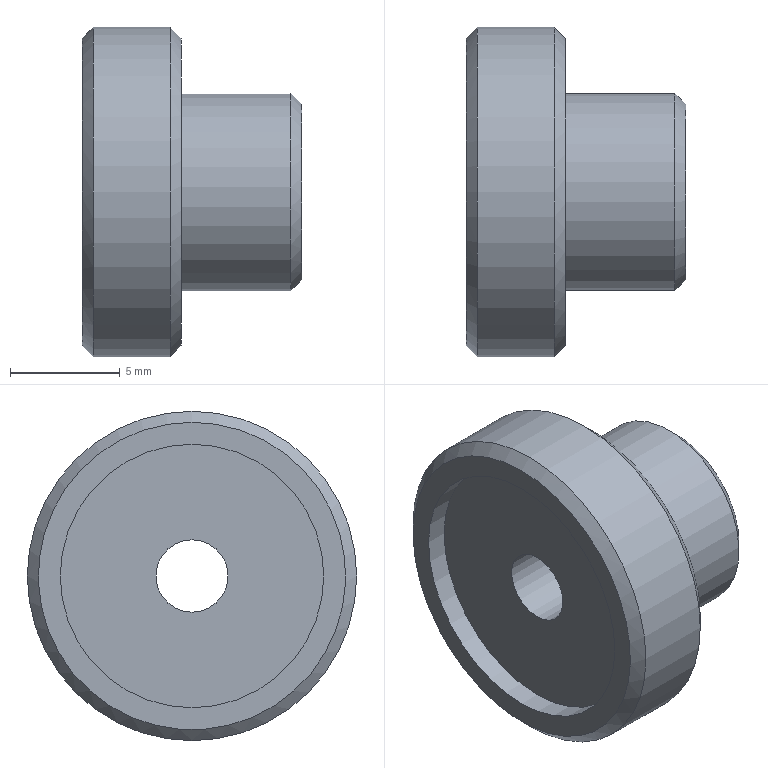Component | NX | 2_KNURLED_NUT | 1 solid | 11 faces | box 10 x 15 x 15 mm | volume 940 mm3 | plane 4 | cylinder 4 | cone 3 | commonest cylinder face diameters 15 x1 9 x1 3.3 x1 12 x1
STEP:
#1=CARTESIAN_POINT('',(0.,0.,0.));
#2=DIRECTION('',(0.,0.,1.));
#3=DIRECTION('',(1.,0.,0.));
#4=AXIS2_PLACEMENT_3D('',#1,#2,#3);
#5=CARTESIAN_POINT('',(-76.584,-174.206,-245.219));
#6=VERTEX_POINT('',#5);
#7=CARTESIAN_POINT('',(-76.584,-174.206,-238.219));
#8=DIRECTION('',(1.,0.,0.));
#9=DIRECTION('',(0.,0.,-1.));
#10=AXIS2_PLACEMENT_3D('',#7,#8,#9);
#11=CIRCLE('',#10,7.);
#12=CARTESIAN_POINT('',(-76.584,-174.206,-238.219));
#13=DIRECTION('',(1.,0.,0.));
#14=DIRECTION('',(0.,0.,-1.));
#15=AXIS2_PLACEMENT_3D('',#12,#13,#14);
#16=PLANE('',#15);
#17=CARTESIAN_POINT('',(0.,0.));
#18=DIRECTION('',(1.,0.));
#19=AXIS2_PLACEMENT_2D('',#17,#18);
#20=CIRCLE('',#19,7.);
#21=(GEOMETRIC_REPRESENTATION_CONTEXT(2)PARAMETRIC_REPRESENTATION_CONTEXT()REPRESENTATION_CONTEXT('',''));
#22=DEFINITIONAL_REPRESENTATION('',(#20),#21);
#23=PCURVE('',#16,#22);
#24=CARTESIAN_POINT('',(-77.084,-174.206,-238.219));
#25=DIRECTION('',(-1.,0.,0.));
#26=DIRECTION('',(0.,0.,1.));
#27=AXIS2_PLACEMENT_3D('',#24,#25,#26);
#28=CONICAL_SURFACE('',#27,7.5,0.7854);
#29=CARTESIAN_POINT('',(9.425,-0.5));
#30=DIRECTION('',(-1.,0.));
#31=VECTOR('',#30,1.);
#32=LINE('',#29,#31);
#33=(GEOMETRIC_REPRESENTATION_CONTEXT(2)PARAMETRIC_REPRESENTATION_CONTEXT()REPRESENTATION_CONTEXT('',''));
#34=DEFINITIONAL_REPRESENTATION('',(#32),#33);
#35=PCURVE('',#28,#34);
#36=SURFACE_CURVE('',#11,(#23,#35),.PCURVE_S1.);
#37=EDGE_CURVE('',#6,#6,#36,.T.);
#38=ORIENTED_EDGE('',*,*,#37,.T.);
#39=EDGE_LOOP('',(#38));
#40=FACE_BOUND('',#39,.T.);
#41=CARTESIAN_POINT('',(-76.584,-174.206,-242.719));
#42=VERTEX_POINT('',#41);
#43=CARTESIAN_POINT('',(-76.584,-174.206,-238.219));
#44=DIRECTION('',(1.,0.,0.));
#45=DIRECTION('',(0.,0.,-1.));
#46=AXIS2_PLACEMENT_3D('',#43,#44,#45);
#47=CIRCLE('',#46,4.5);
#48=CARTESIAN_POINT('',(0.,0.));
#49=DIRECTION('',(1.,0.));
#50=AXIS2_PLACEMENT_2D('',#48,#49);
#51=CIRCLE('',#50,4.5);
#52=(GEOMETRIC_REPRESENTATION_CONTEXT(2)PARAMETRIC_REPRESENTATION_CONTEXT()REPRESENTATION_CONTEXT('',''));
#53=DEFINITIONAL_REPRESENTATION('',(#51),#52);
#54=PCURVE('',#16,#53);
#55=CARTESIAN_POINT('',(-76.584,-174.206,-238.219));
#56=DIRECTION('',(1.,0.,0.));
#57=DIRECTION('',(0.,0.,-1.));
#58=AXIS2_PLACEMENT_3D('',#55,#56,#57);
#59=CYLINDRICAL_SURFACE('',#58,4.5);
#60=CARTESIAN_POINT('',(0.,0.));
#61=DIRECTION('',(1.,0.));
#62=VECTOR('',#61,1.);
#63=LINE('',#60,#62);
#64=(GEOMETRIC_REPRESENTATION_CONTEXT(2)PARAMETRIC_REPRESENTATION_CONTEXT()REPRESENTATION_CONTEXT('',''));
#65=DEFINITIONAL_REPRESENTATION('',(#63),#64);
#66=PCURVE('',#59,#65);
#67=SURFACE_CURVE('',#47,(#54,#66),.PCURVE_S1.);
#68=EDGE_CURVE('',#42,#42,#67,.T.);
#69=ORIENTED_EDGE('',*,*,#68,.F.);
#70=EDGE_LOOP('',(#69));
#71=FACE_BOUND('',#70,.T.);
#72=ADVANCED_FACE('',(#40,#71),#16,.T.);
#73=CARTESIAN_POINT('',(-81.084,-174.206,-244.219));
#74=VERTEX_POINT('',#73);
#75=CARTESIAN_POINT('',(-81.084,-174.206,-238.219));
#76=DIRECTION('',(1.,0.,0.));
#77=DIRECTION('',(0.,0.,-1.));
#78=AXIS2_PLACEMENT_3D('',#75,#76,#77);
#79=CIRCLE('',#78,6.);
#80=CARTESIAN_POINT('',(-81.084,-174.206,-238.219));
#81=DIRECTION('',(-1.,0.,0.));
#82=DIRECTION('',(0.,0.,1.));
#83=AXIS2_PLACEMENT_3D('',#80,#81,#82);
#84=PLANE('',#83);
#85=CARTESIAN_POINT('',(-6.,0.));
#86=CARTESIAN_POINT('',(-6.,10.392));
#87=CARTESIAN_POINT('',(3.,5.196));
#88=CARTESIAN_POINT('',(12.,0.));
#89=CARTESIAN_POINT('',(3.,-5.196));
#90=CARTESIAN_POINT('',(-6.,-10.392));
#91=CARTESIAN_POINT('',(-6.,0.));
#92=(BOUNDED_CURVE()B_SPLINE_CURVE(2,(#85,#86,#87,#88,#89,#90,#91),.UNSPECIFIED.,.T.,.F.)B_SPLINE_CURVE_WITH_KNOTS((1,2,2,2,2,1),(-2.094,0.,2.094,4.189,6.283,8.378),.UNSPECIFIED.)CURVE()GEOMETRIC_REPRESENTATION_ITEM()RATIONAL_B_SPLINE_CURVE((1.,0.5,1.,0.5,1.,0.5,1.))REPRESENTATION_ITEM(''));
#93=(GEOMETRIC_REPRESENTATION_CONTEXT(2)PARAMETRIC_REPRESENTATION_CONTEXT()REPRESENTATION_CONTEXT('',''));
#94=DEFINITIONAL_REPRESENTATION('',(#92),#93);
#95=PCURVE('',#84,#94);
#96=CARTESIAN_POINT('',(-81.084,-174.206,-238.219));
#97=DIRECTION('',(1.,0.,0.));
#98=DIRECTION('',(0.,0.,-1.));
#99=AXIS2_PLACEMENT_3D('',#96,#97,#98);
#100=CYLINDRICAL_SURFACE('',#99,6.);
#101=CARTESIAN_POINT('',(0.,0.));
#102=DIRECTION('',(1.,0.));
#103=VECTOR('',#102,1.);
#104=LINE('',#101,#103);
#105=(GEOMETRIC_REPRESENTATION_CONTEXT(2)PARAMETRIC_REPRESENTATION_CONTEXT()REPRESENTATION_CONTEXT('',''));
#106=DEFINITIONAL_REPRESENTATION('',(#104),#105);
#107=PCURVE('',#100,#106);
#108=SURFACE_CURVE('',#79,(#95,#107),.PCURVE_S1.);
#109=EDGE_CURVE('',#74,#74,#108,.T.);
#110=ORIENTED_EDGE('',*,*,#109,.T.);
#111=EDGE_LOOP('',(#110));
#112=FACE_BOUND('',#111,.T.);
#113=CARTESIAN_POINT('',(-81.084,-174.206,-231.219));
#114=VERTEX_POINT('',#113);
#115=CARTESIAN_POINT('',(-81.084,-174.206,-238.219));
#116=DIRECTION('',(-1.,0.,0.));
#117=DIRECTION('',(0.,0.,1.));
#118=AXIS2_PLACEMENT_3D('',#115,#116,#117);
#119=CIRCLE('',#118,7.);
#120=CARTESIAN_POINT('',(0.,0.));
#121=DIRECTION('',(1.,0.));
#122=AXIS2_PLACEMENT_2D('',#120,#121);
#123=CIRCLE('',#122,7.);
#124=(GEOMETRIC_REPRESENTATION_CONTEXT(2)PARAMETRIC_REPRESENTATION_CONTEXT()REPRESENTATION_CONTEXT('',''));
#125=DEFINITIONAL_REPRESENTATION('',(#123),#124);
#126=PCURVE('',#84,#125);
#127=CARTESIAN_POINT('',(-80.584,-174.206,-238.219));
#128=DIRECTION('',(1.,0.,0.));
#129=DIRECTION('',(0.,0.,-1.));
#130=AXIS2_PLACEMENT_3D('',#127,#128,#129);
#131=CONICAL_SURFACE('',#130,7.5,0.7854);
#132=CARTESIAN_POINT('',(9.425,-0.5));
#133=DIRECTION('',(-1.,0.));
#134=VECTOR('',#133,1.);
#135=LINE('',#132,#134);
#136=(GEOMETRIC_REPRESENTATION_CONTEXT(2)PARAMETRIC_REPRESENTATION_CONTEXT()REPRESENTATION_CONTEXT('',''));
#137=DEFINITIONAL_REPRESENTATION('',(#135),#136);
#138=PCURVE('',#131,#137);
#139=SURFACE_CURVE('',#119,(#126,#138),.PCURVE_S1.);
#140=EDGE_CURVE('',#114,#114,#139,.T.);
#141=ORIENTED_EDGE('',*,*,#140,.T.);
#142=EDGE_LOOP('',(#141));
#143=FACE_BOUND('',#142,.T.);
#144=ADVANCED_FACE('',(#112,#143),#84,.T.);
#145=CARTESIAN_POINT('',(-80.584,-174.206,-230.719));
#146=VERTEX_POINT('',#145);
#147=CARTESIAN_POINT('',(-80.584,-174.206,-245.719));
#148=VERTEX_POINT('',#147);
#149=CARTESIAN_POINT('',(-80.584,-174.206,-238.219));
#150=DIRECTION('',(1.,0.,0.));
#151=DIRECTION('',(0.,0.,1.));
#152=AXIS2_PLACEMENT_3D('',#149,#150,#151);
#153=CIRCLE('',#152,7.5);
#154=CARTESIAN_POINT('',(-81.084,-174.206,-238.219));
#155=DIRECTION('',(1.,0.,0.));
#156=DIRECTION('',(0.,0.,-1.));
#157=AXIS2_PLACEMENT_3D('',#154,#155,#156);
#158=CYLINDRICAL_SURFACE('',#157,7.5);
#159=CARTESIAN_POINT('',(3.142,0.5));
#160=DIRECTION('',(1.,0.));
#161=VECTOR('',#160,1.);
#162=LINE('',#159,#161);
#163=(GEOMETRIC_REPRESENTATION_CONTEXT(2)PARAMETRIC_REPRESENTATION_CONTEXT()REPRESENTATION_CONTEXT('',''));
#164=DEFINITIONAL_REPRESENTATION('',(#162),#163);
#165=PCURVE('',#158,#164);
#166=CARTESIAN_POINT('',(3.142,0.));
#167=DIRECTION('',(1.,0.));
#168=VECTOR('',#167,1.);
#169=LINE('',#166,#168);
#170=(GEOMETRIC_REPRESENTATION_CONTEXT(2)PARAMETRIC_REPRESENTATION_CONTEXT()REPRESENTATION_CONTEXT('',''));
#171=DEFINITIONAL_REPRESENTATION('',(#169),#170);
#172=PCURVE('',#131,#171);
#173=SURFACE_CURVE('',#153,(#165,#172),.PCURVE_S1.);
#174=EDGE_CURVE('',#146,#148,#173,.T.);
#175=ORIENTED_EDGE('',*,*,#174,.T.);
#176=CARTESIAN_POINT('',(-77.084,-174.206,-245.719));
#177=VERTEX_POINT('',#176);
#178=CARTESIAN_POINT('',(-80.584,-174.206,-245.719));
#179=CARTESIAN_POINT('',(-77.084,-174.206,-245.719));
#180=B_SPLINE_CURVE_WITH_KNOTS('',1,(#178,#179),.UNSPECIFIED.,.F.,.F.,(2,2),(0.5,4.),.PIECEWISE_BEZIER_KNOTS.);
#181=CARTESIAN_POINT('',(6.283,0.));
#182=DIRECTION('',(0.,1.));
#183=VECTOR('',#182,1.);
#184=LINE('',#181,#183);
#185=(GEOMETRIC_REPRESENTATION_CONTEXT(2)PARAMETRIC_REPRESENTATION_CONTEXT()REPRESENTATION_CONTEXT('',''));
#186=DEFINITIONAL_REPRESENTATION('',(#184),#185);
#187=PCURVE('',#158,#186);
#188=CARTESIAN_POINT('',(0.,0.));
#189=DIRECTION('',(0.,1.));
#190=VECTOR('',#189,1.);
#191=LINE('',#188,#190);
#192=(GEOMETRIC_REPRESENTATION_CONTEXT(2)PARAMETRIC_REPRESENTATION_CONTEXT()REPRESENTATION_CONTEXT('',''));
#193=DEFINITIONAL_REPRESENTATION('',(#191),#192);
#194=PCURVE('',#158,#193);
#195=SEAM_CURVE('',#180,(#187,#194),.PCURVE_S1.);
#196=EDGE_CURVE('',#148,#177,#195,.T.);
#197=ORIENTED_EDGE('',*,*,#196,.T.);
#198=CARTESIAN_POINT('',(-77.084,-174.206,-238.219));
#199=DIRECTION('',(-1.,0.,0.));
#200=DIRECTION('',(0.,0.,-1.));
#201=AXIS2_PLACEMENT_3D('',#198,#199,#200);
#202=CIRCLE('',#201,7.5);
#203=CARTESIAN_POINT('',(6.283,4.));
#204=DIRECTION('',(-1.,0.));
#205=VECTOR('',#204,1.);
#206=LINE('',#203,#205);
#207=(GEOMETRIC_REPRESENTATION_CONTEXT(2)PARAMETRIC_REPRESENTATION_CONTEXT()REPRESENTATION_CONTEXT('',''));
#208=DEFINITIONAL_REPRESENTATION('',(#206),#207);
#209=PCURVE('',#158,#208);
#210=CARTESIAN_POINT('',(3.142,0.));
#211=DIRECTION('',(1.,0.));
#212=VECTOR('',#211,1.);
#213=LINE('',#210,#212);
#214=(GEOMETRIC_REPRESENTATION_CONTEXT(2)PARAMETRIC_REPRESENTATION_CONTEXT()REPRESENTATION_CONTEXT('',''));
#215=DEFINITIONAL_REPRESENTATION('',(#213),#214);
#216=PCURVE('',#28,#215);
#217=SURFACE_CURVE('',#202,(#209,#216),.PCURVE_S1.);
#218=EDGE_CURVE('',#177,#177,#217,.T.);
#219=ORIENTED_EDGE('',*,*,#218,.T.);
#220=ORIENTED_EDGE('',*,*,#196,.F.);
#221=CARTESIAN_POINT('',(-80.584,-174.206,-238.219));
#222=DIRECTION('',(1.,0.,0.));
#223=DIRECTION('',(0.,0.,1.));
#224=AXIS2_PLACEMENT_3D('',#221,#222,#223);
#225=CIRCLE('',#224,7.5);
#226=CARTESIAN_POINT('',(-3.142,0.5));
#227=DIRECTION('',(1.,0.));
#228=VECTOR('',#227,1.);
#229=LINE('',#226,#228);
#230=(GEOMETRIC_REPRESENTATION_CONTEXT(2)PARAMETRIC_REPRESENTATION_CONTEXT()REPRESENTATION_CONTEXT('',''));
#231=DEFINITIONAL_REPRESENTATION('',(#229),#230);
#232=PCURVE('',#158,#231);
#233=CARTESIAN_POINT('',(3.142,0.));
#234=DIRECTION('',(1.,0.));
#235=VECTOR('',#234,1.);
#236=LINE('',#233,#235);
#237=(GEOMETRIC_REPRESENTATION_CONTEXT(2)PARAMETRIC_REPRESENTATION_CONTEXT()REPRESENTATION_CONTEXT('',''));
#238=DEFINITIONAL_REPRESENTATION('',(#236),#237);
#239=PCURVE('',#131,#238);
#240=SURFACE_CURVE('',#225,(#232,#239),.PCURVE_S1.);
#241=EDGE_CURVE('',#148,#146,#240,.T.);
#242=ORIENTED_EDGE('',*,*,#241,.T.);
#243=EDGE_LOOP('',(#175,#197,#219,#220,#242));
#244=FACE_BOUND('',#243,.T.);
#245=ADVANCED_FACE('',(#244),#158,.T.);
#246=CARTESIAN_POINT('',(-71.084,-174.206,-242.219));
#247=VERTEX_POINT('',#246);
#248=CARTESIAN_POINT('',(-71.084,-174.206,-238.219));
#249=DIRECTION('',(1.,0.,0.));
#250=DIRECTION('',(0.,0.,-1.));
#251=AXIS2_PLACEMENT_3D('',#248,#249,#250);
#252=CIRCLE('',#251,4.);
#253=CARTESIAN_POINT('',(-71.084,-174.206,-238.219));
#254=DIRECTION('',(1.,0.,0.));
#255=DIRECTION('',(0.,0.,-1.));
#256=AXIS2_PLACEMENT_3D('',#253,#254,#255);
#257=PLANE('',#256);
#258=CARTESIAN_POINT('',(0.,0.));
#259=DIRECTION('',(1.,0.));
#260=AXIS2_PLACEMENT_2D('',#258,#259);
#261=CIRCLE('',#260,4.);
#262=(GEOMETRIC_REPRESENTATION_CONTEXT(2)PARAMETRIC_REPRESENTATION_CONTEXT()REPRESENTATION_CONTEXT('',''));
#263=DEFINITIONAL_REPRESENTATION('',(#261),#262);
#264=PCURVE('',#257,#263);
#265=CARTESIAN_POINT('',(-71.584,-174.206,-238.219));
#266=DIRECTION('',(-1.,0.,0.));
#267=DIRECTION('',(0.,0.,1.));
#268=AXIS2_PLACEMENT_3D('',#265,#266,#267);
#269=CONICAL_SURFACE('',#268,4.5,0.7854);
#270=CARTESIAN_POINT('',(9.425,-0.5));
#271=DIRECTION('',(-1.,0.));
#272=VECTOR('',#271,1.);
#273=LINE('',#270,#272);
#274=(GEOMETRIC_REPRESENTATION_CONTEXT(2)PARAMETRIC_REPRESENTATION_CONTEXT()REPRESENTATION_CONTEXT('',''));
#275=DEFINITIONAL_REPRESENTATION('',(#273),#274);
#276=PCURVE('',#269,#275);
#277=SURFACE_CURVE('',#252,(#264,#276),.PCURVE_S1.);
#278=EDGE_CURVE('',#247,#247,#277,.T.);
#279=ORIENTED_EDGE('',*,*,#278,.T.);
#280=EDGE_LOOP('',(#279));
#281=FACE_BOUND('',#280,.T.);
#282=CARTESIAN_POINT('',(-71.084,-174.206,-236.569));
#283=VERTEX_POINT('',#282);
#284=CARTESIAN_POINT('',(-71.084,-174.206,-238.219));
#285=DIRECTION('',(-1.,0.,0.));
#286=DIRECTION('',(0.,0.,1.));
#287=AXIS2_PLACEMENT_3D('',#284,#285,#286);
#288=CIRCLE('',#287,1.65);
#289=CARTESIAN_POINT('',(-1.65,0.));
#290=CARTESIAN_POINT('',(-1.65,2.858));
#291=CARTESIAN_POINT('',(0.825,1.429));
#292=CARTESIAN_POINT('',(3.3,0.));
#293=CARTESIAN_POINT('',(0.825,-1.429));
#294=CARTESIAN_POINT('',(-1.65,-2.858));
#295=CARTESIAN_POINT('',(-1.65,0.));
#296=(BOUNDED_CURVE()B_SPLINE_CURVE(2,(#289,#290,#291,#292,#293,#294,#295),.UNSPECIFIED.,.T.,.F.)B_SPLINE_CURVE_WITH_KNOTS((1,2,2,2,2,1),(-2.094,0.,2.094,4.189,6.283,8.378),.UNSPECIFIED.)CURVE()GEOMETRIC_REPRESENTATION_ITEM()RATIONAL_B_SPLINE_CURVE((1.,0.5,1.,0.5,1.,0.5,1.))REPRESENTATION_ITEM(''));
#297=(GEOMETRIC_REPRESENTATION_CONTEXT(2)PARAMETRIC_REPRESENTATION_CONTEXT()REPRESENTATION_CONTEXT('',''));
#298=DEFINITIONAL_REPRESENTATION('',(#296),#297);
#299=PCURVE('',#257,#298);
#300=CARTESIAN_POINT('',(-71.084,-174.206,-238.219));
#301=DIRECTION('',(-1.,0.,0.));
#302=DIRECTION('',(0.,0.,1.));
#303=AXIS2_PLACEMENT_3D('',#300,#301,#302);
#304=CYLINDRICAL_SURFACE('',#303,1.65);
#305=CARTESIAN_POINT('',(0.,0.));
#306=DIRECTION('',(1.,0.));
#307=VECTOR('',#306,1.);
#308=LINE('',#305,#307);
#309=(GEOMETRIC_REPRESENTATION_CONTEXT(2)PARAMETRIC_REPRESENTATION_CONTEXT()REPRESENTATION_CONTEXT('',''));
#310=DEFINITIONAL_REPRESENTATION('',(#308),#309);
#311=PCURVE('',#304,#310);
#312=SURFACE_CURVE('',#288,(#299,#311),.PCURVE_S1.);
#313=EDGE_CURVE('',#283,#283,#312,.T.);
#314=ORIENTED_EDGE('',*,*,#313,.T.);
#315=EDGE_LOOP('',(#314));
#316=FACE_BOUND('',#315,.T.);
#317=ADVANCED_FACE('',(#281,#316),#257,.T.);
#318=CARTESIAN_POINT('',(-71.584,-174.206,-242.719));
#319=VERTEX_POINT('',#318);
#320=CARTESIAN_POINT('',(-71.584,-174.206,-238.219));
#321=DIRECTION('',(-1.,0.,0.));
#322=DIRECTION('',(0.,0.,-1.));
#323=AXIS2_PLACEMENT_3D('',#320,#321,#322);
#324=CIRCLE('',#323,4.5);
#325=CARTESIAN_POINT('',(6.283,5.));
#326=DIRECTION('',(-1.,0.));
#327=VECTOR('',#326,1.);
#328=LINE('',#325,#327);
#329=(GEOMETRIC_REPRESENTATION_CONTEXT(2)PARAMETRIC_REPRESENTATION_CONTEXT()REPRESENTATION_CONTEXT('',''));
#330=DEFINITIONAL_REPRESENTATION('',(#328),#329);
#331=PCURVE('',#59,#330);
#332=CARTESIAN_POINT('',(3.142,0.));
#333=DIRECTION('',(1.,0.));
#334=VECTOR('',#333,1.);
#335=LINE('',#332,#334);
#336=(GEOMETRIC_REPRESENTATION_CONTEXT(2)PARAMETRIC_REPRESENTATION_CONTEXT()REPRESENTATION_CONTEXT('',''));
#337=DEFINITIONAL_REPRESENTATION('',(#335),#336);
#338=PCURVE('',#269,#337);
#339=SURFACE_CURVE('',#324,(#331,#338),.PCURVE_S1.);
#340=EDGE_CURVE('',#319,#319,#339,.T.);
#341=ORIENTED_EDGE('',*,*,#340,.T.);
#342=CARTESIAN_POINT('',(-76.584,-174.206,-242.719));
#343=CARTESIAN_POINT('',(-71.584,-174.206,-242.719));
#344=B_SPLINE_CURVE_WITH_KNOTS('',1,(#342,#343),.UNSPECIFIED.,.F.,.F.,(2,2),(0.,5.),.PIECEWISE_BEZIER_KNOTS.);
#345=CARTESIAN_POINT('',(0.,0.));
#346=DIRECTION('',(0.,1.));
#347=VECTOR('',#346,1.);
#348=LINE('',#345,#347);
#349=(GEOMETRIC_REPRESENTATION_CONTEXT(2)PARAMETRIC_REPRESENTATION_CONTEXT()REPRESENTATION_CONTEXT('',''));
#350=DEFINITIONAL_REPRESENTATION('',(#348),#349);
#351=PCURVE('',#59,#350);
#352=CARTESIAN_POINT('',(6.283,0.));
#353=DIRECTION('',(0.,1.));
#354=VECTOR('',#353,1.);
#355=LINE('',#352,#354);
#356=(GEOMETRIC_REPRESENTATION_CONTEXT(2)PARAMETRIC_REPRESENTATION_CONTEXT()REPRESENTATION_CONTEXT('',''));
#357=DEFINITIONAL_REPRESENTATION('',(#355),#356);
#358=PCURVE('',#59,#357);
#359=SEAM_CURVE('',#344,(#351,#358),.PCURVE_S1.);
#360=EDGE_CURVE('',#42,#319,#359,.T.);
#361=ORIENTED_EDGE('',*,*,#360,.F.);
#362=ORIENTED_EDGE('',*,*,#68,.T.);
#363=ORIENTED_EDGE('',*,*,#360,.T.);
#364=EDGE_LOOP('',(#341,#361,#362,#363));
#365=FACE_BOUND('',#364,.T.);
#366=ADVANCED_FACE('',(#365),#59,.T.);
#367=CARTESIAN_POINT('',(-80.084,-174.206,-236.569));
#368=VERTEX_POINT('',#367);
#369=CARTESIAN_POINT('',(-80.084,-174.206,-239.869));
#370=VERTEX_POINT('',#369);
#371=CARTESIAN_POINT('',(-80.084,-174.206,-238.219));
#372=DIRECTION('',(-1.,0.,0.));
#373=DIRECTION('',(0.,0.,-1.));
#374=AXIS2_PLACEMENT_3D('',#371,#372,#373);
#375=CIRCLE('',#374,1.65);
#376=CARTESIAN_POINT('',(-3.142,9.));
#377=DIRECTION('',(1.,0.));
#378=VECTOR('',#377,1.);
#379=LINE('',#376,#378);
#380=(GEOMETRIC_REPRESENTATION_CONTEXT(2)PARAMETRIC_REPRESENTATION_CONTEXT()REPRESENTATION_CONTEXT('',''));
#381=DEFINITIONAL_REPRESENTATION('',(#379),#380);
#382=PCURVE('',#304,#381);
#383=CARTESIAN_POINT('',(-80.084,-174.206,-238.219));
#384=DIRECTION('',(1.,0.,0.));
#385=DIRECTION('',(0.,0.,-1.));
#386=AXIS2_PLACEMENT_3D('',#383,#384,#385);
#387=PLANE('',#386);
#388=CARTESIAN_POINT('',(1.65,0.));
#389=CARTESIAN_POINT('',(1.65,-2.858));
#390=CARTESIAN_POINT('',(-0.825,-1.429));
#391=CARTESIAN_POINT('',(-3.3,-0.));
#392=CARTESIAN_POINT('',(-0.825,1.429));
#393=CARTESIAN_POINT('',(1.65,2.858));
#394=CARTESIAN_POINT('',(1.65,0.));
#395=(BOUNDED_CURVE()B_SPLINE_CURVE(2,(#388,#389,#390,#391,#392,#393,#394),.UNSPECIFIED.,.T.,.F.)B_SPLINE_CURVE_WITH_KNOTS((1,2,2,2,2,1),(-2.094,0.,2.094,4.189,6.283,8.378),.UNSPECIFIED.)CURVE()GEOMETRIC_REPRESENTATION_ITEM()RATIONAL_B_SPLINE_CURVE((1.,0.5,1.,0.5,1.,0.5,1.))REPRESENTATION_ITEM(''));
#396=(GEOMETRIC_REPRESENTATION_CONTEXT(2)PARAMETRIC_REPRESENTATION_CONTEXT()REPRESENTATION_CONTEXT('',''));
#397=DEFINITIONAL_REPRESENTATION('',(#395),#396);
#398=PCURVE('',#387,#397);
#399=SURFACE_CURVE('',#375,(#382,#398),.PCURVE_S1.);
#400=EDGE_CURVE('',#368,#370,#399,.T.);
#401=ORIENTED_EDGE('',*,*,#400,.F.);
#402=CARTESIAN_POINT('',(-71.084,-174.206,-236.569));
#403=CARTESIAN_POINT('',(-80.084,-174.206,-236.569));
#404=B_SPLINE_CURVE_WITH_KNOTS('',1,(#402,#403),.UNSPECIFIED.,.F.,.F.,(2,2),(0.,9.),.PIECEWISE_BEZIER_KNOTS.);
#405=CARTESIAN_POINT('',(0.,0.));
#406=DIRECTION('',(0.,1.));
#407=VECTOR('',#406,1.);
#408=LINE('',#405,#407);
#409=(GEOMETRIC_REPRESENTATION_CONTEXT(2)PARAMETRIC_REPRESENTATION_CONTEXT()REPRESENTATION_CONTEXT('',''));
#410=DEFINITIONAL_REPRESENTATION('',(#408),#409);
#411=PCURVE('',#304,#410);
#412=CARTESIAN_POINT('',(6.283,0.));
#413=DIRECTION('',(0.,1.));
#414=VECTOR('',#413,1.);
#415=LINE('',#412,#414);
#416=(GEOMETRIC_REPRESENTATION_CONTEXT(2)PARAMETRIC_REPRESENTATION_CONTEXT()REPRESENTATION_CONTEXT('',''));
#417=DEFINITIONAL_REPRESENTATION('',(#415),#416);
#418=PCURVE('',#304,#417);
#419=SEAM_CURVE('',#404,(#411,#418),.PCURVE_S1.);
#420=EDGE_CURVE('',#283,#368,#419,.T.);
#421=ORIENTED_EDGE('',*,*,#420,.F.);
#422=ORIENTED_EDGE('',*,*,#313,.T.);
#423=ORIENTED_EDGE('',*,*,#420,.T.);
#424=CARTESIAN_POINT('',(-80.084,-174.206,-238.219));
#425=DIRECTION('',(-1.,0.,0.));
#426=DIRECTION('',(0.,0.,-1.));
#427=AXIS2_PLACEMENT_3D('',#424,#425,#426);
#428=CIRCLE('',#427,1.65);
#429=CARTESIAN_POINT('',(3.142,9.));
#430=DIRECTION('',(1.,0.));
#431=VECTOR('',#430,1.);
#432=LINE('',#429,#431);
#433=(GEOMETRIC_REPRESENTATION_CONTEXT(2)PARAMETRIC_REPRESENTATION_CONTEXT()REPRESENTATION_CONTEXT('',''));
#434=DEFINITIONAL_REPRESENTATION('',(#432),#433);
#435=PCURVE('',#304,#434);
#436=CARTESIAN_POINT('',(1.65,0.));
#437=CARTESIAN_POINT('',(1.65,-2.858));
#438=CARTESIAN_POINT('',(-0.825,-1.429));
#439=CARTESIAN_POINT('',(-3.3,-0.));
#440=CARTESIAN_POINT('',(-0.825,1.429));
#441=CARTESIAN_POINT('',(1.65,2.858));
#442=CARTESIAN_POINT('',(1.65,0.));
#443=(BOUNDED_CURVE()B_SPLINE_CURVE(2,(#436,#437,#438,#439,#440,#441,#442),.UNSPECIFIED.,.T.,.F.)B_SPLINE_CURVE_WITH_KNOTS((1,2,2,2,2,1),(-2.094,0.,2.094,4.189,6.283,8.378),.UNSPECIFIED.)CURVE()GEOMETRIC_REPRESENTATION_ITEM()RATIONAL_B_SPLINE_CURVE((1.,0.5,1.,0.5,1.,0.5,1.))REPRESENTATION_ITEM(''));
#444=(GEOMETRIC_REPRESENTATION_CONTEXT(2)PARAMETRIC_REPRESENTATION_CONTEXT()REPRESENTATION_CONTEXT('',''));
#445=DEFINITIONAL_REPRESENTATION('',(#443),#444);
#446=PCURVE('',#387,#445);
#447=SURFACE_CURVE('',#428,(#435,#446),.PCURVE_S1.);
#448=EDGE_CURVE('',#370,#368,#447,.T.);
#449=ORIENTED_EDGE('',*,*,#448,.F.);
#450=EDGE_LOOP('',(#401,#421,#422,#423,#449));
#451=FACE_BOUND('',#450,.F.);
#452=ADVANCED_FACE('',(#451),#304,.F.);
#453=ORIENTED_EDGE('',*,*,#140,.F.);
#454=CARTESIAN_POINT('',(-81.084,-174.206,-231.219));
#455=CARTESIAN_POINT('',(-80.584,-174.206,-230.719));
#456=B_SPLINE_CURVE_WITH_KNOTS('',1,(#454,#455),.UNSPECIFIED.,.F.,.F.,(2,2),(-0.7071,0.),.PIECEWISE_BEZIER_KNOTS.);
#457=CARTESIAN_POINT('',(9.425,0.));
#458=DIRECTION('',(0.,1.));
#459=VECTOR('',#458,1.);
#460=LINE('',#457,#459);
#461=(GEOMETRIC_REPRESENTATION_CONTEXT(2)PARAMETRIC_REPRESENTATION_CONTEXT()REPRESENTATION_CONTEXT('',''));
#462=DEFINITIONAL_REPRESENTATION('',(#460),#461);
#463=PCURVE('',#131,#462);
#464=CARTESIAN_POINT('',(3.142,0.));
#465=DIRECTION('',(0.,1.));
#466=VECTOR('',#465,1.);
#467=LINE('',#464,#466);
#468=(GEOMETRIC_REPRESENTATION_CONTEXT(2)PARAMETRIC_REPRESENTATION_CONTEXT()REPRESENTATION_CONTEXT('',''));
#469=DEFINITIONAL_REPRESENTATION('',(#467),#468);
#470=PCURVE('',#131,#469);
#471=SEAM_CURVE('',#456,(#463,#470),.PCURVE_S1.);
#472=EDGE_CURVE('',#114,#146,#471,.T.);
#473=ORIENTED_EDGE('',*,*,#472,.T.);
#474=ORIENTED_EDGE('',*,*,#241,.F.);
#475=ORIENTED_EDGE('',*,*,#174,.F.);
#476=ORIENTED_EDGE('',*,*,#472,.F.);
#477=EDGE_LOOP('',(#453,#473,#474,#475,#476));
#478=FACE_BOUND('',#477,.T.);
#479=ADVANCED_FACE('',(#478),#131,.T.);
#480=ORIENTED_EDGE('',*,*,#37,.F.);
#481=CARTESIAN_POINT('',(-76.584,-174.206,-245.219));
#482=CARTESIAN_POINT('',(-77.084,-174.206,-245.719));
#483=B_SPLINE_CURVE_WITH_KNOTS('',1,(#481,#482),.UNSPECIFIED.,.F.,.F.,(2,2),(-0.7071,0.),.PIECEWISE_BEZIER_KNOTS.);
#484=CARTESIAN_POINT('',(9.425,0.));
#485=DIRECTION('',(0.,1.));
#486=VECTOR('',#485,1.);
#487=LINE('',#484,#486);
#488=(GEOMETRIC_REPRESENTATION_CONTEXT(2)PARAMETRIC_REPRESENTATION_CONTEXT()REPRESENTATION_CONTEXT('',''));
#489=DEFINITIONAL_REPRESENTATION('',(#487),#488);
#490=PCURVE('',#28,#489);
#491=CARTESIAN_POINT('',(3.142,0.));
#492=DIRECTION('',(0.,1.));
#493=VECTOR('',#492,1.);
#494=LINE('',#491,#493);
#495=(GEOMETRIC_REPRESENTATION_CONTEXT(2)PARAMETRIC_REPRESENTATION_CONTEXT()REPRESENTATION_CONTEXT('',''));
#496=DEFINITIONAL_REPRESENTATION('',(#494),#495);
#497=PCURVE('',#28,#496);
#498=SEAM_CURVE('',#483,(#490,#497),.PCURVE_S1.);
#499=EDGE_CURVE('',#6,#177,#498,.T.);
#500=ORIENTED_EDGE('',*,*,#499,.T.);
#501=ORIENTED_EDGE('',*,*,#218,.F.);
#502=ORIENTED_EDGE('',*,*,#499,.F.);
#503=EDGE_LOOP('',(#480,#500,#501,#502));
#504=FACE_BOUND('',#503,.T.);
#505=ADVANCED_FACE('',(#504),#28,.T.);
#506=ORIENTED_EDGE('',*,*,#278,.F.);
#507=CARTESIAN_POINT('',(-71.084,-174.206,-242.219));
#508=CARTESIAN_POINT('',(-71.584,-174.206,-242.719));
#509=B_SPLINE_CURVE_WITH_KNOTS('',1,(#507,#508),.UNSPECIFIED.,.F.,.F.,(2,2),(-0.7071,0.),.PIECEWISE_BEZIER_KNOTS.);
#510=CARTESIAN_POINT('',(9.425,0.));
#511=DIRECTION('',(0.,1.));
#512=VECTOR('',#511,1.);
#513=LINE('',#510,#512);
#514=(GEOMETRIC_REPRESENTATION_CONTEXT(2)PARAMETRIC_REPRESENTATION_CONTEXT()REPRESENTATION_CONTEXT('',''));
#515=DEFINITIONAL_REPRESENTATION('',(#513),#514);
#516=PCURVE('',#269,#515);
#517=CARTESIAN_POINT('',(3.142,0.));
#518=DIRECTION('',(0.,1.));
#519=VECTOR('',#518,1.);
#520=LINE('',#517,#519);
#521=(GEOMETRIC_REPRESENTATION_CONTEXT(2)PARAMETRIC_REPRESENTATION_CONTEXT()REPRESENTATION_CONTEXT('',''));
#522=DEFINITIONAL_REPRESENTATION('',(#520),#521);
#523=PCURVE('',#269,#522);
#524=SEAM_CURVE('',#509,(#516,#523),.PCURVE_S1.);
#525=EDGE_CURVE('',#247,#319,#524,.T.);
#526=ORIENTED_EDGE('',*,*,#525,.T.);
#527=ORIENTED_EDGE('',*,*,#340,.F.);
#528=ORIENTED_EDGE('',*,*,#525,.F.);
#529=EDGE_LOOP('',(#506,#526,#527,#528));
#530=FACE_BOUND('',#529,.T.);
#531=ADVANCED_FACE('',(#530),#269,.T.);
#532=CARTESIAN_POINT('',(-80.084,-174.206,-244.219));
#533=VERTEX_POINT('',#532);
#534=CARTESIAN_POINT('',(-80.084,-174.206,-238.219));
#535=DIRECTION('',(1.,0.,0.));
#536=DIRECTION('',(0.,0.,-1.));
#537=AXIS2_PLACEMENT_3D('',#534,#535,#536);
#538=CIRCLE('',#537,6.);
#539=CARTESIAN_POINT('',(0.,0.));
#540=DIRECTION('',(1.,0.));
#541=AXIS2_PLACEMENT_2D('',#539,#540);
#542=CIRCLE('',#541,6.);
#543=(GEOMETRIC_REPRESENTATION_CONTEXT(2)PARAMETRIC_REPRESENTATION_CONTEXT()REPRESENTATION_CONTEXT('',''));
#544=DEFINITIONAL_REPRESENTATION('',(#542),#543);
#545=PCURVE('',#387,#544);
#546=CARTESIAN_POINT('',(0.,1.));
#547=DIRECTION('',(1.,0.));
#548=VECTOR('',#547,1.);
#549=LINE('',#546,#548);
#550=(GEOMETRIC_REPRESENTATION_CONTEXT(2)PARAMETRIC_REPRESENTATION_CONTEXT()REPRESENTATION_CONTEXT('',''));
#551=DEFINITIONAL_REPRESENTATION('',(#549),#550);
#552=PCURVE('',#100,#551);
#553=SURFACE_CURVE('',#538,(#545,#552),.PCURVE_S1.);
#554=EDGE_CURVE('',#533,#533,#553,.T.);
#555=ORIENTED_EDGE('',*,*,#554,.F.);
#556=EDGE_LOOP('',(#555));
#557=FACE_BOUND('',#556,.T.);
#558=ORIENTED_EDGE('',*,*,#448,.F.);
#559=ORIENTED_EDGE('',*,*,#400,.F.);
#560=EDGE_LOOP('',(#558,#559));
#561=FACE_BOUND('',#560,.T.);
#562=ADVANCED_FACE('',(#557,#561),#387,.F.);
#563=ORIENTED_EDGE('',*,*,#554,.F.);
#564=CARTESIAN_POINT('',(-81.084,-174.206,-244.219));
#565=CARTESIAN_POINT('',(-80.084,-174.206,-244.219));
#566=B_SPLINE_CURVE_WITH_KNOTS('',1,(#564,#565),.UNSPECIFIED.,.F.,.F.,(2,2),(0.,1.),.PIECEWISE_BEZIER_KNOTS.);
#567=CARTESIAN_POINT('',(0.,0.));
#568=DIRECTION('',(0.,1.));
#569=VECTOR('',#568,1.);
#570=LINE('',#567,#569);
#571=(GEOMETRIC_REPRESENTATION_CONTEXT(2)PARAMETRIC_REPRESENTATION_CONTEXT()REPRESENTATION_CONTEXT('',''));
#572=DEFINITIONAL_REPRESENTATION('',(#570),#571);
#573=PCURVE('',#100,#572);
#574=CARTESIAN_POINT('',(6.283,0.));
#575=DIRECTION('',(0.,1.));
#576=VECTOR('',#575,1.);
#577=LINE('',#574,#576);
#578=(GEOMETRIC_REPRESENTATION_CONTEXT(2)PARAMETRIC_REPRESENTATION_CONTEXT()REPRESENTATION_CONTEXT('',''));
#579=DEFINITIONAL_REPRESENTATION('',(#577),#578);
#580=PCURVE('',#100,#579);
#581=SEAM_CURVE('',#566,(#573,#580),.PCURVE_S1.);
#582=EDGE_CURVE('',#74,#533,#581,.T.);
#583=ORIENTED_EDGE('',*,*,#582,.F.);
#584=ORIENTED_EDGE('',*,*,#109,.T.);
#585=ORIENTED_EDGE('',*,*,#582,.T.);
#586=EDGE_LOOP('',(#563,#583,#584,#585));
#587=FACE_BOUND('',#586,.F.);
#588=ADVANCED_FACE('',(#587),#100,.F.);
#589=CLOSED_SHELL('',(#72,#144,#245,#317,#366,#452,#479,#505,#531,#562,#588));
#590=MANIFOLD_SOLID_BREP('',#589);
#591=(LENGTH_UNIT()NAMED_UNIT(*)SI_UNIT(.MILLI.,.METRE.));
#592=UNCERTAINTY_MEASURE_WITH_UNIT(LENGTH_MEASURE(0.00001),#591,'','');
#593=(NAMED_UNIT(*)PLANE_ANGLE_UNIT()SI_UNIT($,.RADIAN.));
#594=(NAMED_UNIT(*)SI_UNIT($,.STERADIAN.)SOLID_ANGLE_UNIT());
#595=(GEOMETRIC_REPRESENTATION_CONTEXT(3)GLOBAL_UNCERTAINTY_ASSIGNED_CONTEXT((#592))GLOBAL_UNIT_ASSIGNED_CONTEXT((#591,#593,#594))REPRESENTATION_CONTEXT('',''));
#596=ADVANCED_BREP_SHAPE_REPRESENTATION('',(#4,#590),#595);